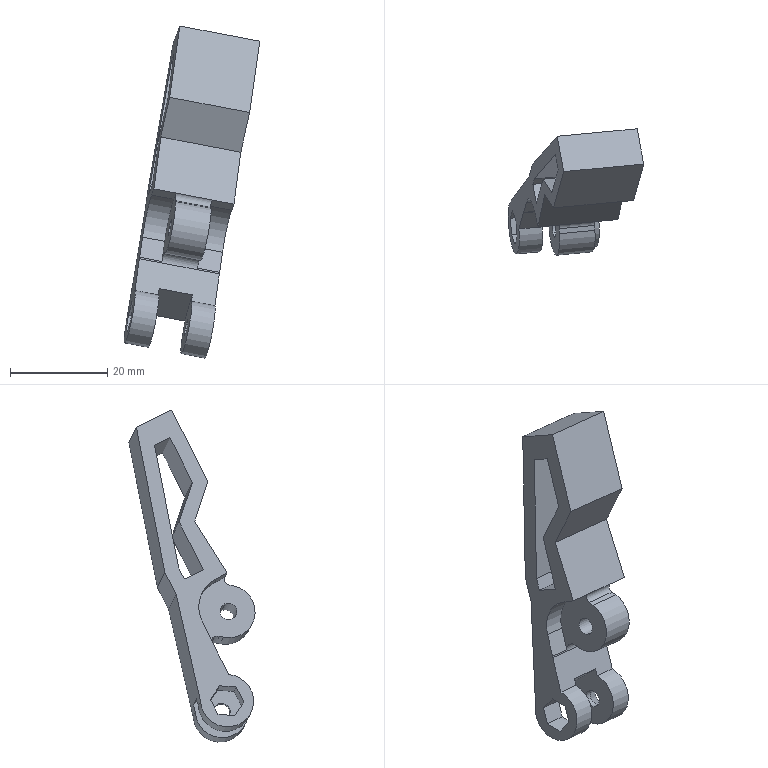Component | SolidWorks | Pinza1-16-SW-1 | 1 solid | 49 faces | box 27.9 x 25.99 x 68.4 mm | volume 7478 mm3 | plane 35 | cylinder 12 | cone 2 | commonest cylinder face diameters 3.293 x2 3.5 x2 3.498 x2 10.997 x2 13.2 x2 2.2 x1 11 x1
build123d program:
from build123d import *

# Parameters (mm, degrees)
SKETCH4_R           = 1.75
SKETCH4_R_2         = 1.749
BOSS_EXTRUDE1_DEPTH = 16.84
CUT_EXTRUDE1_DEPTH  = 4.68
CUT_EXTRUDE2_DEPTH  = 5
SKETCH7_W           = 44.257
SKETCH7_H           = 7
CUT_EXTRUDE3_DEPTH  = 27.5
CUT_EXTRUDE4_DEPTH  = 3.5
CHAMFER3_SIZE       = 3.5
CHAMFER3_SIZE2      = 1.783


with BuildPart() as part:
    # Sketch4 → Boss-Extrude1 (new body)
    with BuildSketch(Plane.XY):
        with BuildLine():
            Line((-365.53, 297.456), (-335.814, 306.057))
            Line((-335.814, 306.057), (-330.641, 306.086))
            Line((-330.641, 306.086), (-308.449, 311.782))
            ThreePointArc((-308.449, 311.782), (-300.97, 305.089), (-310.943, 303.964))
            Line((-310.943, 303.964), (-318.344, 303.908))
            ThreePointArc((-318.344, 303.908), (-319.734, 302.934), (-319.524, 301.249))
            Line((-319.524, 301.249), (-318.996, 300.574))
            ThreePointArc((-318.996, 300.574), (-319.939, 292.853), (-327.66, 293.796))
            Line((-327.66, 293.796), (-328.304, 294.619))
            ThreePointArc((-328.304, 294.619), (-329.188, 295.041), (-330.058, 294.59))
            Line((-330.058, 294.59), (-342.685, 295.623))
            Line((-342.685, 295.623), (-348.887, 289.351))
            Line((-348.887, 289.351), (-365.484, 289.257))
            Line((-365.484, 289.257), (-365.53, 297.456))
        make_face()
        with Locations((-323.328, 297.185)):
            Circle(SKETCH4_R, mode=Mode.SUBTRACT)
        with Locations((-306.209, 306.76)):
            Circle(SKETCH4_R_2, mode=Mode.SUBTRACT)
        Polygon((-360.506, 295.818), (-335.384, 303.089), (-332.827, 303.104), (-332.802, 298.649), (-343.932, 298.586), (-350.134, 292.314), (-360.486, 292.255), align=None, mode=Mode.SUBTRACT)
    extrude(amount=BOSS_EXTRUDE1_DEPTH)

    # Sketch5 → Cut-Extrude1 (cut)
    with BuildSketch(Plane.XY.offset(16.84)):
        with BuildLine():
            Line((-310.943, 303.964), (-323.328, 303.785))
            ThreePointArc((-323.328, 303.785), (-327.995, 301.852), (-329.928, 297.185))
            Line((-329.928, 297.185), (-330.058, 294.59))
            Line((-330.058, 294.59), (-328.322, 292.87))
            ThreePointArc((-328.322, 292.87), (-322.903, 290.599), (-317.82, 293.548))
            Line((-317.82, 293.548), (-310.943, 303.964))
        make_face()
    cut_extrude1 = extrude(amount=-CUT_EXTRUDE1_DEPTH, mode=Mode.SUBTRACT)

    # Mirror1: Cut-Extrude1 across plane
    add(cut_extrude1.mirror(Plane.XY.offset(8.42)), mode=Mode.SUBTRACT)

    # Sketch6 → Cut-Extrude2 (cut)
    with BuildSketch(Plane(origin=(0, 0, 0), x_dir=(-1, 0, 0), z_dir=(0, 0, -1))):
        Polygon((304.5, 309.773), (302.745, 306.787), (304.454, 303.774), (307.918, 303.747), (309.673, 306.734), (307.964, 309.747), align=None)
    extrude(amount=-CUT_EXTRUDE2_DEPTH, mode=Mode.SUBTRACT)

    # Sketch7 → Cut-Extrude3 (cut, symmetric)
    with BuildSketch(Plane(origin=(-94.143, 366.787, 0), x_dir=(0.9686, 0.2486, 0), z_dir=(-0.2486, 0.9686, 0))):
        with Locations((-200.704, -8.42)):
            Rectangle(SKETCH7_W, SKETCH7_H)
    extrude(amount=CUT_EXTRUDE3_DEPTH, both=True, mode=Mode.SUBTRACT)

    # Sketch8 → Cut-Extrude4 (cut, symmetric)
    with BuildSketch(Plane.XY.offset(8.42)):
        Polygon((-309.977, 311.39), (-312.417, 303.953), (-305.778, 299.179), (-297.83, 303.723), (-297.83, 313.028), (-306.949, 313.3), align=None)
    extrude(amount=CUT_EXTRUDE4_DEPTH, both=True, mode=Mode.SUBTRACT)

    # Chamfer3
    chamfer3_edges = [part.edges().sort_by_distance(p)[0] for p in [
        (-307.958, 306.76, 16.84),
    ]]
    chamfer3_side = [part.faces().sort_by_distance(p)[0] for p in [
        (-307.958, 306.76, 14.38),
    ]]
    chamfer(chamfer3_edges, length=CHAMFER3_SIZE, length2=CHAMFER3_SIZE2, reference=chamfer3_side[0])


solid = part.part

# Placed as in the assembly
solid = solid.moved(Location((86.786, -448.707, 745.13), (-153.738, 78.061, 127.106)))